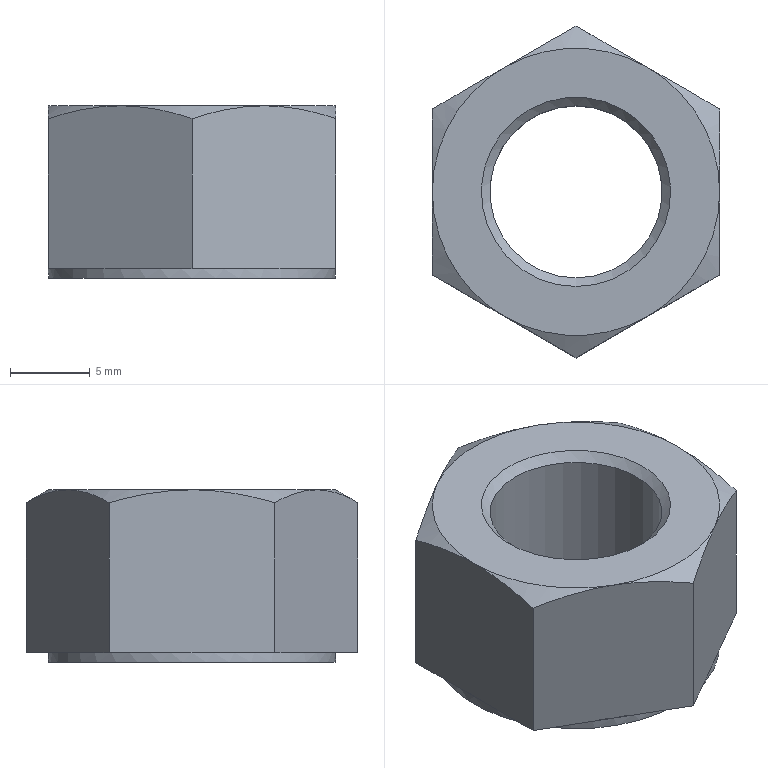Component | NX | GB-T6171_T-2000_M12X1_5 | 1 solid | 23 faces | volume 2017 mm3 | plane 14 | cone 7 | cylinder 2 | commonest cylinder face diameters 18 x1 10.782 x1